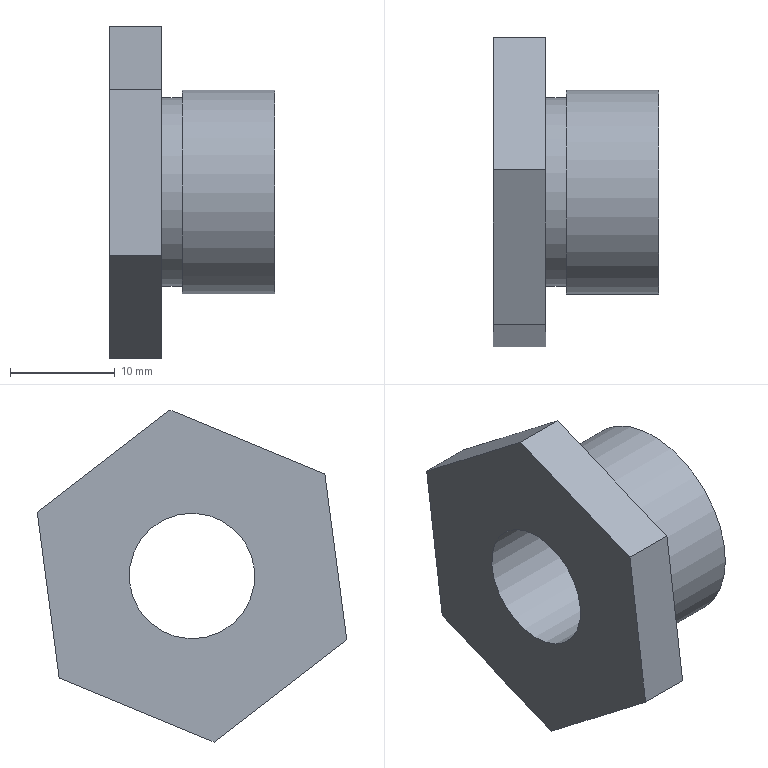Component | NX | LOCK_SLEEVE | 1 solid | 13 faces | box 15.82 x 29.58 x 31.72 mm | volume 4679 mm3 | plane 10 | cylinder 3 | commonest cylinder face diameters 19.5 x1 12 x1 18 x1
STEP:
#1=CARTESIAN_POINT('',(0.,0.,0.));
#2=DIRECTION('',(0.,0.,1.));
#3=DIRECTION('',(1.,0.,0.));
#4=AXIS2_PLACEMENT_3D('',#1,#2,#3);
#5=CARTESIAN_POINT('',(83.182,-9.011,-3.723));
#6=VERTEX_POINT('',#5);
#7=CARTESIAN_POINT('',(83.182,0.,0.));
#8=DIRECTION('',(1.,0.,0.));
#9=DIRECTION('',(0.,-0.9242,-0.3818));
#10=AXIS2_PLACEMENT_3D('',#7,#8,#9);
#11=CIRCLE('',#10,9.75);
#12=CARTESIAN_POINT('',(92.,0.,0.));
#13=DIRECTION('',(-1.,0.,0.));
#14=DIRECTION('',(0.,0.9242,0.3818));
#15=AXIS2_PLACEMENT_3D('',#12,#13,#14);
#16=CYLINDRICAL_SURFACE('',#15,9.75);
#17=CARTESIAN_POINT('',(9.425,8.818));
#18=DIRECTION('',(-1.,0.));
#19=VECTOR('',#18,1.);
#20=LINE('',#17,#19);
#21=(GEOMETRIC_REPRESENTATION_CONTEXT(2)PARAMETRIC_REPRESENTATION_CONTEXT()REPRESENTATION_CONTEXT('',''));
#22=DEFINITIONAL_REPRESENTATION('',(#20),#21);
#23=PCURVE('',#16,#22);
#24=CARTESIAN_POINT('',(83.182,0.,0.));
#25=DIRECTION('',(1.,0.,0.));
#26=DIRECTION('',(0.,-0.9242,-0.3818));
#27=AXIS2_PLACEMENT_3D('',#24,#25,#26);
#28=PLANE('',#27);
#29=CARTESIAN_POINT('',(0.,0.));
#30=DIRECTION('',(1.,0.));
#31=AXIS2_PLACEMENT_2D('',#29,#30);
#32=CIRCLE('',#31,9.75);
#33=(GEOMETRIC_REPRESENTATION_CONTEXT(2)PARAMETRIC_REPRESENTATION_CONTEXT()REPRESENTATION_CONTEXT('',''));
#34=DEFINITIONAL_REPRESENTATION('',(#32),#33);
#35=PCURVE('',#28,#34);
#36=SURFACE_CURVE('',#11,(#23,#35),.PCURVE_S1.);
#37=EDGE_CURVE('',#6,#6,#36,.T.);
#38=ORIENTED_EDGE('',*,*,#37,.T.);
#39=CARTESIAN_POINT('',(92.,-9.011,-3.723));
#40=VERTEX_POINT('',#39);
#41=CARTESIAN_POINT('',(92.,-9.011,-3.723));
#42=CARTESIAN_POINT('',(83.182,-9.011,-3.723));
#43=B_SPLINE_CURVE_WITH_KNOTS('',1,(#41,#42),.UNSPECIFIED.,.F.,.F.,(2,2),(0.,8.818),.PIECEWISE_BEZIER_KNOTS.);
#44=CARTESIAN_POINT('',(3.142,0.));
#45=DIRECTION('',(0.,1.));
#46=VECTOR('',#45,1.);
#47=LINE('',#44,#46);
#48=(GEOMETRIC_REPRESENTATION_CONTEXT(2)PARAMETRIC_REPRESENTATION_CONTEXT()REPRESENTATION_CONTEXT('',''));
#49=DEFINITIONAL_REPRESENTATION('',(#47),#48);
#50=PCURVE('',#16,#49);
#51=CARTESIAN_POINT('',(9.425,0.));
#52=DIRECTION('',(0.,1.));
#53=VECTOR('',#52,1.);
#54=LINE('',#51,#53);
#55=(GEOMETRIC_REPRESENTATION_CONTEXT(2)PARAMETRIC_REPRESENTATION_CONTEXT()REPRESENTATION_CONTEXT('',''));
#56=DEFINITIONAL_REPRESENTATION('',(#54),#55);
#57=PCURVE('',#16,#56);
#58=SEAM_CURVE('',#43,(#50,#57),.PCURVE_S1.);
#59=EDGE_CURVE('',#40,#6,#58,.T.);
#60=ORIENTED_EDGE('',*,*,#59,.F.);
#61=CARTESIAN_POINT('',(92.,0.,0.));
#62=DIRECTION('',(1.,0.,0.));
#63=DIRECTION('',(0.,-0.9242,-0.3818));
#64=AXIS2_PLACEMENT_3D('',#61,#62,#63);
#65=CIRCLE('',#64,9.75);
#66=CARTESIAN_POINT('',(9.425,0.));
#67=DIRECTION('',(-1.,0.));
#68=VECTOR('',#67,1.);
#69=LINE('',#66,#68);
#70=(GEOMETRIC_REPRESENTATION_CONTEXT(2)PARAMETRIC_REPRESENTATION_CONTEXT()REPRESENTATION_CONTEXT('',''));
#71=DEFINITIONAL_REPRESENTATION('',(#69),#70);
#72=PCURVE('',#16,#71);
#73=CARTESIAN_POINT('',(92.,0.,0.));
#74=DIRECTION('',(1.,0.,0.));
#75=DIRECTION('',(0.,-0.9242,-0.3818));
#76=AXIS2_PLACEMENT_3D('',#73,#74,#75);
#77=PLANE('',#76);
#78=CARTESIAN_POINT('',(0.,0.));
#79=DIRECTION('',(1.,0.));
#80=AXIS2_PLACEMENT_2D('',#78,#79);
#81=CIRCLE('',#80,9.75);
#82=(GEOMETRIC_REPRESENTATION_CONTEXT(2)PARAMETRIC_REPRESENTATION_CONTEXT()REPRESENTATION_CONTEXT('',''));
#83=DEFINITIONAL_REPRESENTATION('',(#81),#82);
#84=PCURVE('',#77,#83);
#85=SURFACE_CURVE('',#65,(#72,#84),.PCURVE_S1.);
#86=EDGE_CURVE('',#40,#40,#85,.T.);
#87=ORIENTED_EDGE('',*,*,#86,.F.);
#88=ORIENTED_EDGE('',*,*,#59,.T.);
#89=EDGE_LOOP('',(#38,#60,#87,#88));
#90=FACE_BOUND('',#89,.T.);
#91=ADVANCED_FACE('',(#90),#16,.T.);
#92=CARTESIAN_POINT('',(92.,-5.545,-2.291));
#93=VERTEX_POINT('',#92);
#94=CARTESIAN_POINT('',(92.,0.,0.));
#95=DIRECTION('',(-1.,0.,0.));
#96=DIRECTION('',(0.,-0.9242,-0.3818));
#97=AXIS2_PLACEMENT_3D('',#94,#95,#96);
#98=CIRCLE('',#97,6.);
#99=CARTESIAN_POINT('',(6.,0.));
#100=CARTESIAN_POINT('',(6.,-10.392));
#101=CARTESIAN_POINT('',(-3.,-5.196));
#102=CARTESIAN_POINT('',(-12.,-0.));
#103=CARTESIAN_POINT('',(-3.,5.196));
#104=CARTESIAN_POINT('',(6.,10.392));
#105=CARTESIAN_POINT('',(6.,0.));
#106=(BOUNDED_CURVE()B_SPLINE_CURVE(2,(#99,#100,#101,#102,#103,#104,#105),.UNSPECIFIED.,.T.,.F.)B_SPLINE_CURVE_WITH_KNOTS((1,2,2,2,2,1),(-2.094,0.,2.094,4.189,6.283,8.378),.UNSPECIFIED.)CURVE()GEOMETRIC_REPRESENTATION_ITEM()RATIONAL_B_SPLINE_CURVE((1.,0.5,1.,0.5,1.,0.5,1.))REPRESENTATION_ITEM(''));
#107=(GEOMETRIC_REPRESENTATION_CONTEXT(2)PARAMETRIC_REPRESENTATION_CONTEXT()REPRESENTATION_CONTEXT('',''));
#108=DEFINITIONAL_REPRESENTATION('',(#106),#107);
#109=PCURVE('',#77,#108);
#110=CARTESIAN_POINT('',(102.182,0.,0.));
#111=DIRECTION('',(-1.,0.,0.));
#112=DIRECTION('',(0.,0.9242,0.3818));
#113=AXIS2_PLACEMENT_3D('',#110,#111,#112);
#114=CYLINDRICAL_SURFACE('',#113,6.);
#115=CARTESIAN_POINT('',(3.142,10.182));
#116=DIRECTION('',(1.,0.));
#117=VECTOR('',#116,1.);
#118=LINE('',#115,#117);
#119=(GEOMETRIC_REPRESENTATION_CONTEXT(2)PARAMETRIC_REPRESENTATION_CONTEXT()REPRESENTATION_CONTEXT('',''));
#120=DEFINITIONAL_REPRESENTATION('',(#118),#119);
#121=PCURVE('',#114,#120);
#122=SURFACE_CURVE('',#98,(#109,#121),.PCURVE_S1.);
#123=EDGE_CURVE('',#93,#93,#122,.T.);
#124=ORIENTED_EDGE('',*,*,#123,.T.);
#125=EDGE_LOOP('',(#124));
#126=FACE_BOUND('',#125,.T.);
#127=ORIENTED_EDGE('',*,*,#86,.T.);
#128=EDGE_LOOP('',(#127));
#129=FACE_BOUND('',#128,.T.);
#130=ADVANCED_FACE('',(#126,#129),#77,.T.);
#131=CARTESIAN_POINT('',(81.182,14.788,6.11));
#132=VERTEX_POINT('',#131);
#133=CARTESIAN_POINT('',(81.182,2.103,15.861));
#134=VERTEX_POINT('',#133);
#135=CARTESIAN_POINT('',(81.182,14.788,6.11));
#136=DIRECTION('',(0.,-0.7928,0.6095));
#137=VECTOR('',#136,1.);
#138=LINE('',#135,#137);
#139=CARTESIAN_POINT('',(76.182,14.788,6.11));
#140=DIRECTION('',(0.,0.6095,0.7928));
#141=DIRECTION('',(0.,-0.7928,0.6095));
#142=AXIS2_PLACEMENT_3D('',#139,#140,#141);
#143=PLANE('',#142);
#144=CARTESIAN_POINT('',(0.,5.));
#145=DIRECTION('',(1.,0.));
#146=VECTOR('',#145,1.);
#147=LINE('',#144,#146);
#148=(GEOMETRIC_REPRESENTATION_CONTEXT(2)PARAMETRIC_REPRESENTATION_CONTEXT()REPRESENTATION_CONTEXT('',''));
#149=DEFINITIONAL_REPRESENTATION('',(#147),#148);
#150=PCURVE('',#143,#149);
#151=CARTESIAN_POINT('',(81.182,0.,0.));
#152=DIRECTION('',(1.,0.,0.));
#153=DIRECTION('',(0.,-0.9242,-0.3818));
#154=AXIS2_PLACEMENT_3D('',#151,#152,#153);
#155=PLANE('',#154);
#156=CARTESIAN_POINT('',(-16.,0.));
#157=DIRECTION('',(0.5,-0.866));
#158=VECTOR('',#157,1.);
#159=LINE('',#156,#158);
#160=(GEOMETRIC_REPRESENTATION_CONTEXT(2)PARAMETRIC_REPRESENTATION_CONTEXT()REPRESENTATION_CONTEXT('',''));
#161=DEFINITIONAL_REPRESENTATION('',(#159),#160);
#162=PCURVE('',#155,#161);
#163=SURFACE_CURVE('',#138,(#150,#162),.PCURVE_S1.);
#164=EDGE_CURVE('',#132,#134,#163,.T.);
#165=ORIENTED_EDGE('',*,*,#164,.F.);
#166=CARTESIAN_POINT('',(76.182,14.788,6.11));
#167=VERTEX_POINT('',#166);
#168=CARTESIAN_POINT('',(76.182,14.788,6.11));
#169=DIRECTION('',(1.,0.,0.));
#170=VECTOR('',#169,1.);
#171=LINE('',#168,#170);
#172=CARTESIAN_POINT('',(0.,0.));
#173=DIRECTION('',(0.,1.));
#174=VECTOR('',#173,1.);
#175=LINE('',#172,#174);
#176=(GEOMETRIC_REPRESENTATION_CONTEXT(2)PARAMETRIC_REPRESENTATION_CONTEXT()REPRESENTATION_CONTEXT('',''));
#177=DEFINITIONAL_REPRESENTATION('',(#175),#176);
#178=PCURVE('',#143,#177);
#179=CARTESIAN_POINT('',(76.182,12.685,-9.752));
#180=DIRECTION('',(0.,0.9913,-0.1314));
#181=DIRECTION('',(0.,0.1314,0.9913));
#182=AXIS2_PLACEMENT_3D('',#179,#180,#181);
#183=PLANE('',#182);
#184=CARTESIAN_POINT('',(16.,0.));
#185=DIRECTION('',(0.,1.));
#186=VECTOR('',#185,1.);
#187=LINE('',#184,#186);
#188=(GEOMETRIC_REPRESENTATION_CONTEXT(2)PARAMETRIC_REPRESENTATION_CONTEXT()REPRESENTATION_CONTEXT('',''));
#189=DEFINITIONAL_REPRESENTATION('',(#187),#188);
#190=PCURVE('',#183,#189);
#191=SURFACE_CURVE('',#171,(#178,#190),.PCURVE_S1.);
#192=EDGE_CURVE('',#167,#132,#191,.T.);
#193=ORIENTED_EDGE('',*,*,#192,.F.);
#194=CARTESIAN_POINT('',(76.182,2.103,15.861));
#195=VERTEX_POINT('',#194);
#196=CARTESIAN_POINT('',(76.182,14.788,6.11));
#197=DIRECTION('',(0.,-0.7928,0.6095));
#198=VECTOR('',#197,1.);
#199=LINE('',#196,#198);
#200=CARTESIAN_POINT('',(0.,0.));
#201=DIRECTION('',(1.,0.));
#202=VECTOR('',#201,1.);
#203=LINE('',#200,#202);
#204=(GEOMETRIC_REPRESENTATION_CONTEXT(2)PARAMETRIC_REPRESENTATION_CONTEXT()REPRESENTATION_CONTEXT('',''));
#205=DEFINITIONAL_REPRESENTATION('',(#203),#204);
#206=PCURVE('',#143,#205);
#207=CARTESIAN_POINT('',(76.182,0.,0.));
#208=DIRECTION('',(1.,0.,0.));
#209=DIRECTION('',(0.,-0.9242,-0.3818));
#210=AXIS2_PLACEMENT_3D('',#207,#208,#209);
#211=PLANE('',#210);
#212=CARTESIAN_POINT('',(-16.,0.));
#213=DIRECTION('',(0.5,-0.866));
#214=VECTOR('',#213,1.);
#215=LINE('',#212,#214);
#216=(GEOMETRIC_REPRESENTATION_CONTEXT(2)PARAMETRIC_REPRESENTATION_CONTEXT()REPRESENTATION_CONTEXT('',''));
#217=DEFINITIONAL_REPRESENTATION('',(#215),#216);
#218=PCURVE('',#211,#217);
#219=SURFACE_CURVE('',#199,(#206,#218),.PCURVE_S1.);
#220=EDGE_CURVE('',#167,#195,#219,.T.);
#221=ORIENTED_EDGE('',*,*,#220,.T.);
#222=CARTESIAN_POINT('',(76.182,2.103,15.861));
#223=DIRECTION('',(1.,0.,0.));
#224=VECTOR('',#223,1.);
#225=LINE('',#222,#224);
#226=CARTESIAN_POINT('',(16.,0.));
#227=DIRECTION('',(0.,1.));
#228=VECTOR('',#227,1.);
#229=LINE('',#226,#228);
#230=(GEOMETRIC_REPRESENTATION_CONTEXT(2)PARAMETRIC_REPRESENTATION_CONTEXT()REPRESENTATION_CONTEXT('',''));
#231=DEFINITIONAL_REPRESENTATION('',(#229),#230);
#232=PCURVE('',#143,#231);
#233=CARTESIAN_POINT('',(76.182,2.103,15.861));
#234=DIRECTION('',(0.,-0.3818,0.9242));
#235=DIRECTION('',(0.,-0.9242,-0.3818));
#236=AXIS2_PLACEMENT_3D('',#233,#234,#235);
#237=PLANE('',#236);
#238=CARTESIAN_POINT('',(0.,0.));
#239=DIRECTION('',(0.,1.));
#240=VECTOR('',#239,1.);
#241=LINE('',#238,#240);
#242=(GEOMETRIC_REPRESENTATION_CONTEXT(2)PARAMETRIC_REPRESENTATION_CONTEXT()REPRESENTATION_CONTEXT('',''));
#243=DEFINITIONAL_REPRESENTATION('',(#241),#242);
#244=PCURVE('',#237,#243);
#245=SURFACE_CURVE('',#225,(#232,#244),.PCURVE_S1.);
#246=EDGE_CURVE('',#195,#134,#245,.T.);
#247=ORIENTED_EDGE('',*,*,#246,.T.);
#248=EDGE_LOOP('',(#165,#193,#221,#247));
#249=FACE_BOUND('',#248,.T.);
#250=ADVANCED_FACE('',(#249),#143,.T.);
#251=CARTESIAN_POINT('',(81.182,-12.685,9.752));
#252=VERTEX_POINT('',#251);
#253=CARTESIAN_POINT('',(81.182,2.103,15.861));
#254=DIRECTION('',(0.,-0.9242,-0.3818));
#255=VECTOR('',#254,1.);
#256=LINE('',#253,#255);
#257=CARTESIAN_POINT('',(0.,5.));
#258=DIRECTION('',(1.,0.));
#259=VECTOR('',#258,1.);
#260=LINE('',#257,#259);
#261=(GEOMETRIC_REPRESENTATION_CONTEXT(2)PARAMETRIC_REPRESENTATION_CONTEXT()REPRESENTATION_CONTEXT('',''));
#262=DEFINITIONAL_REPRESENTATION('',(#260),#261);
#263=PCURVE('',#237,#262);
#264=CARTESIAN_POINT('',(-8.,-13.856));
#265=DIRECTION('',(1.,-0.));
#266=VECTOR('',#265,1.);
#267=LINE('',#264,#266);
#268=(GEOMETRIC_REPRESENTATION_CONTEXT(2)PARAMETRIC_REPRESENTATION_CONTEXT()REPRESENTATION_CONTEXT('',''));
#269=DEFINITIONAL_REPRESENTATION('',(#267),#268);
#270=PCURVE('',#155,#269);
#271=SURFACE_CURVE('',#256,(#263,#270),.PCURVE_S1.);
#272=EDGE_CURVE('',#134,#252,#271,.T.);
#273=ORIENTED_EDGE('',*,*,#272,.F.);
#274=ORIENTED_EDGE('',*,*,#246,.F.);
#275=CARTESIAN_POINT('',(76.182,-12.685,9.752));
#276=VERTEX_POINT('',#275);
#277=CARTESIAN_POINT('',(76.182,2.103,15.861));
#278=DIRECTION('',(0.,-0.9242,-0.3818));
#279=VECTOR('',#278,1.);
#280=LINE('',#277,#279);
#281=CARTESIAN_POINT('',(0.,0.));
#282=DIRECTION('',(1.,0.));
#283=VECTOR('',#282,1.);
#284=LINE('',#281,#283);
#285=(GEOMETRIC_REPRESENTATION_CONTEXT(2)PARAMETRIC_REPRESENTATION_CONTEXT()REPRESENTATION_CONTEXT('',''));
#286=DEFINITIONAL_REPRESENTATION('',(#284),#285);
#287=PCURVE('',#237,#286);
#288=CARTESIAN_POINT('',(-8.,-13.856));
#289=DIRECTION('',(1.,-0.));
#290=VECTOR('',#289,1.);
#291=LINE('',#288,#290);
#292=(GEOMETRIC_REPRESENTATION_CONTEXT(2)PARAMETRIC_REPRESENTATION_CONTEXT()REPRESENTATION_CONTEXT('',''));
#293=DEFINITIONAL_REPRESENTATION('',(#291),#292);
#294=PCURVE('',#211,#293);
#295=SURFACE_CURVE('',#280,(#287,#294),.PCURVE_S1.);
#296=EDGE_CURVE('',#195,#276,#295,.T.);
#297=ORIENTED_EDGE('',*,*,#296,.T.);
#298=CARTESIAN_POINT('',(76.182,-12.685,9.752));
#299=DIRECTION('',(1.,0.,0.));
#300=VECTOR('',#299,1.);
#301=LINE('',#298,#300);
#302=CARTESIAN_POINT('',(16.,0.));
#303=DIRECTION('',(0.,1.));
#304=VECTOR('',#303,1.);
#305=LINE('',#302,#304);
#306=(GEOMETRIC_REPRESENTATION_CONTEXT(2)PARAMETRIC_REPRESENTATION_CONTEXT()REPRESENTATION_CONTEXT('',''));
#307=DEFINITIONAL_REPRESENTATION('',(#305),#306);
#308=PCURVE('',#237,#307);
#309=CARTESIAN_POINT('',(76.182,-12.685,9.752));
#310=DIRECTION('',(0.,-0.9913,0.1314));
#311=DIRECTION('',(0.,-0.1314,-0.9913));
#312=AXIS2_PLACEMENT_3D('',#309,#310,#311);
#313=PLANE('',#312);
#314=CARTESIAN_POINT('',(0.,0.));
#315=DIRECTION('',(0.,1.));
#316=VECTOR('',#315,1.);
#317=LINE('',#314,#316);
#318=(GEOMETRIC_REPRESENTATION_CONTEXT(2)PARAMETRIC_REPRESENTATION_CONTEXT()REPRESENTATION_CONTEXT('',''));
#319=DEFINITIONAL_REPRESENTATION('',(#317),#318);
#320=PCURVE('',#313,#319);
#321=SURFACE_CURVE('',#301,(#308,#320),.PCURVE_S1.);
#322=EDGE_CURVE('',#276,#252,#321,.T.);
#323=ORIENTED_EDGE('',*,*,#322,.T.);
#324=EDGE_LOOP('',(#273,#274,#297,#323));
#325=FACE_BOUND('',#324,.T.);
#326=ADVANCED_FACE('',(#325),#237,.T.);
#327=CARTESIAN_POINT('',(81.182,-14.788,-6.11));
#328=VERTEX_POINT('',#327);
#329=CARTESIAN_POINT('',(81.182,-12.685,9.752));
#330=DIRECTION('',(0.,-0.1314,-0.9913));
#331=VECTOR('',#330,1.);
#332=LINE('',#329,#331);
#333=CARTESIAN_POINT('',(0.,5.));
#334=DIRECTION('',(1.,0.));
#335=VECTOR('',#334,1.);
#336=LINE('',#333,#335);
#337=(GEOMETRIC_REPRESENTATION_CONTEXT(2)PARAMETRIC_REPRESENTATION_CONTEXT()REPRESENTATION_CONTEXT('',''));
#338=DEFINITIONAL_REPRESENTATION('',(#336),#337);
#339=PCURVE('',#313,#338);
#340=CARTESIAN_POINT('',(8.,-13.856));
#341=DIRECTION('',(0.5,0.866));
#342=VECTOR('',#341,1.);
#343=LINE('',#340,#342);
#344=(GEOMETRIC_REPRESENTATION_CONTEXT(2)PARAMETRIC_REPRESENTATION_CONTEXT()REPRESENTATION_CONTEXT('',''));
#345=DEFINITIONAL_REPRESENTATION('',(#343),#344);
#346=PCURVE('',#155,#345);
#347=SURFACE_CURVE('',#332,(#339,#346),.PCURVE_S1.);
#348=EDGE_CURVE('',#252,#328,#347,.T.);
#349=ORIENTED_EDGE('',*,*,#348,.F.);
#350=ORIENTED_EDGE('',*,*,#322,.F.);
#351=CARTESIAN_POINT('',(76.182,-14.788,-6.11));
#352=VERTEX_POINT('',#351);
#353=CARTESIAN_POINT('',(76.182,-12.685,9.752));
#354=DIRECTION('',(0.,-0.1314,-0.9913));
#355=VECTOR('',#354,1.);
#356=LINE('',#353,#355);
#357=CARTESIAN_POINT('',(0.,0.));
#358=DIRECTION('',(1.,0.));
#359=VECTOR('',#358,1.);
#360=LINE('',#357,#359);
#361=(GEOMETRIC_REPRESENTATION_CONTEXT(2)PARAMETRIC_REPRESENTATION_CONTEXT()REPRESENTATION_CONTEXT('',''));
#362=DEFINITIONAL_REPRESENTATION('',(#360),#361);
#363=PCURVE('',#313,#362);
#364=CARTESIAN_POINT('',(8.,-13.856));
#365=DIRECTION('',(0.5,0.866));
#366=VECTOR('',#365,1.);
#367=LINE('',#364,#366);
#368=(GEOMETRIC_REPRESENTATION_CONTEXT(2)PARAMETRIC_REPRESENTATION_CONTEXT()REPRESENTATION_CONTEXT('',''));
#369=DEFINITIONAL_REPRESENTATION('',(#367),#368);
#370=PCURVE('',#211,#369);
#371=SURFACE_CURVE('',#356,(#363,#370),.PCURVE_S1.);
#372=EDGE_CURVE('',#276,#352,#371,.T.);
#373=ORIENTED_EDGE('',*,*,#372,.T.);
#374=CARTESIAN_POINT('',(76.182,-14.788,-6.11));
#375=DIRECTION('',(1.,0.,0.));
#376=VECTOR('',#375,1.);
#377=LINE('',#374,#376);
#378=CARTESIAN_POINT('',(16.,0.));
#379=DIRECTION('',(0.,1.));
#380=VECTOR('',#379,1.);
#381=LINE('',#378,#380);
#382=(GEOMETRIC_REPRESENTATION_CONTEXT(2)PARAMETRIC_REPRESENTATION_CONTEXT()REPRESENTATION_CONTEXT('',''));
#383=DEFINITIONAL_REPRESENTATION('',(#381),#382);
#384=PCURVE('',#313,#383);
#385=CARTESIAN_POINT('',(76.182,-14.788,-6.11));
#386=DIRECTION('',(0.,-0.6095,-0.7928));
#387=DIRECTION('',(0.,0.7928,-0.6095));
#388=AXIS2_PLACEMENT_3D('',#385,#386,#387);
#389=PLANE('',#388);
#390=CARTESIAN_POINT('',(-0.,0.));
#391=DIRECTION('',(0.,1.));
#392=VECTOR('',#391,1.);
#393=LINE('',#390,#392);
#394=(GEOMETRIC_REPRESENTATION_CONTEXT(2)PARAMETRIC_REPRESENTATION_CONTEXT()REPRESENTATION_CONTEXT('',''));
#395=DEFINITIONAL_REPRESENTATION('',(#393),#394);
#396=PCURVE('',#389,#395);
#397=SURFACE_CURVE('',#377,(#384,#396),.PCURVE_S1.);
#398=EDGE_CURVE('',#352,#328,#397,.T.);
#399=ORIENTED_EDGE('',*,*,#398,.T.);
#400=EDGE_LOOP('',(#349,#350,#373,#399));
#401=FACE_BOUND('',#400,.T.);
#402=ADVANCED_FACE('',(#401),#313,.T.);
#403=CARTESIAN_POINT('',(81.182,-2.103,-15.861));
#404=VERTEX_POINT('',#403);
#405=CARTESIAN_POINT('',(81.182,-14.788,-6.11));
#406=DIRECTION('',(0.,0.7928,-0.6095));
#407=VECTOR('',#406,1.);
#408=LINE('',#405,#407);
#409=CARTESIAN_POINT('',(0.,5.));
#410=DIRECTION('',(1.,0.));
#411=VECTOR('',#410,1.);
#412=LINE('',#409,#411);
#413=(GEOMETRIC_REPRESENTATION_CONTEXT(2)PARAMETRIC_REPRESENTATION_CONTEXT()REPRESENTATION_CONTEXT('',''));
#414=DEFINITIONAL_REPRESENTATION('',(#412),#413);
#415=PCURVE('',#389,#414);
#416=CARTESIAN_POINT('',(16.,-0.));
#417=DIRECTION('',(-0.5,0.866));
#418=VECTOR('',#417,1.);
#419=LINE('',#416,#418);
#420=(GEOMETRIC_REPRESENTATION_CONTEXT(2)PARAMETRIC_REPRESENTATION_CONTEXT()REPRESENTATION_CONTEXT('',''));
#421=DEFINITIONAL_REPRESENTATION('',(#419),#420);
#422=PCURVE('',#155,#421);
#423=SURFACE_CURVE('',#408,(#415,#422),.PCURVE_S1.);
#424=EDGE_CURVE('',#328,#404,#423,.T.);
#425=ORIENTED_EDGE('',*,*,#424,.F.);
#426=ORIENTED_EDGE('',*,*,#398,.F.);
#427=CARTESIAN_POINT('',(76.182,-2.103,-15.861));
#428=VERTEX_POINT('',#427);
#429=CARTESIAN_POINT('',(76.182,-14.788,-6.11));
#430=DIRECTION('',(0.,0.7928,-0.6095));
#431=VECTOR('',#430,1.);
#432=LINE('',#429,#431);
#433=CARTESIAN_POINT('',(0.,0.));
#434=DIRECTION('',(1.,0.));
#435=VECTOR('',#434,1.);
#436=LINE('',#433,#435);
#437=(GEOMETRIC_REPRESENTATION_CONTEXT(2)PARAMETRIC_REPRESENTATION_CONTEXT()REPRESENTATION_CONTEXT('',''));
#438=DEFINITIONAL_REPRESENTATION('',(#436),#437);
#439=PCURVE('',#389,#438);
#440=CARTESIAN_POINT('',(16.,-0.));
#441=DIRECTION('',(-0.5,0.866));
#442=VECTOR('',#441,1.);
#443=LINE('',#440,#442);
#444=(GEOMETRIC_REPRESENTATION_CONTEXT(2)PARAMETRIC_REPRESENTATION_CONTEXT()REPRESENTATION_CONTEXT('',''));
#445=DEFINITIONAL_REPRESENTATION('',(#443),#444);
#446=PCURVE('',#211,#445);
#447=SURFACE_CURVE('',#432,(#439,#446),.PCURVE_S1.);
#448=EDGE_CURVE('',#352,#428,#447,.T.);
#449=ORIENTED_EDGE('',*,*,#448,.T.);
#450=CARTESIAN_POINT('',(76.182,-2.103,-15.861));
#451=DIRECTION('',(1.,0.,0.));
#452=VECTOR('',#451,1.);
#453=LINE('',#450,#452);
#454=CARTESIAN_POINT('',(16.,0.));
#455=DIRECTION('',(0.,1.));
#456=VECTOR('',#455,1.);
#457=LINE('',#454,#456);
#458=(GEOMETRIC_REPRESENTATION_CONTEXT(2)PARAMETRIC_REPRESENTATION_CONTEXT()REPRESENTATION_CONTEXT('',''));
#459=DEFINITIONAL_REPRESENTATION('',(#457),#458);
#460=PCURVE('',#389,#459);
#461=CARTESIAN_POINT('',(76.182,-2.103,-15.861));
#462=DIRECTION('',(0.,0.3818,-0.9242));
#463=DIRECTION('',(0.,0.9242,0.3818));
#464=AXIS2_PLACEMENT_3D('',#461,#462,#463);
#465=PLANE('',#464);
#466=CARTESIAN_POINT('',(0.,0.));
#467=DIRECTION('',(0.,1.));
#468=VECTOR('',#467,1.);
#469=LINE('',#466,#468);
#470=(GEOMETRIC_REPRESENTATION_CONTEXT(2)PARAMETRIC_REPRESENTATION_CONTEXT()REPRESENTATION_CONTEXT('',''));
#471=DEFINITIONAL_REPRESENTATION('',(#469),#470);
#472=PCURVE('',#465,#471);
#473=SURFACE_CURVE('',#453,(#460,#472),.PCURVE_S1.);
#474=EDGE_CURVE('',#428,#404,#473,.T.);
#475=ORIENTED_EDGE('',*,*,#474,.T.);
#476=EDGE_LOOP('',(#425,#426,#449,#475));
#477=FACE_BOUND('',#476,.T.);
#478=ADVANCED_FACE('',(#477),#389,.T.);
#479=CARTESIAN_POINT('',(81.182,12.685,-9.752));
#480=VERTEX_POINT('',#479);
#481=CARTESIAN_POINT('',(81.182,-2.103,-15.861));
#482=DIRECTION('',(0.,0.9242,0.3818));
#483=VECTOR('',#482,1.);
#484=LINE('',#481,#483);
#485=CARTESIAN_POINT('',(0.,5.));
#486=DIRECTION('',(1.,0.));
#487=VECTOR('',#486,1.);
#488=LINE('',#485,#487);
#489=(GEOMETRIC_REPRESENTATION_CONTEXT(2)PARAMETRIC_REPRESENTATION_CONTEXT()REPRESENTATION_CONTEXT('',''));
#490=DEFINITIONAL_REPRESENTATION('',(#488),#489);
#491=PCURVE('',#465,#490);
#492=CARTESIAN_POINT('',(8.,13.856));
#493=DIRECTION('',(-1.,0.));
#494=VECTOR('',#493,1.);
#495=LINE('',#492,#494);
#496=(GEOMETRIC_REPRESENTATION_CONTEXT(2)PARAMETRIC_REPRESENTATION_CONTEXT()REPRESENTATION_CONTEXT('',''));
#497=DEFINITIONAL_REPRESENTATION('',(#495),#496);
#498=PCURVE('',#155,#497);
#499=SURFACE_CURVE('',#484,(#491,#498),.PCURVE_S1.);
#500=EDGE_CURVE('',#404,#480,#499,.T.);
#501=ORIENTED_EDGE('',*,*,#500,.F.);
#502=ORIENTED_EDGE('',*,*,#474,.F.);
#503=CARTESIAN_POINT('',(76.182,12.685,-9.752));
#504=VERTEX_POINT('',#503);
#505=CARTESIAN_POINT('',(76.182,-2.103,-15.861));
#506=DIRECTION('',(0.,0.9242,0.3818));
#507=VECTOR('',#506,1.);
#508=LINE('',#505,#507);
#509=CARTESIAN_POINT('',(0.,0.));
#510=DIRECTION('',(1.,0.));
#511=VECTOR('',#510,1.);
#512=LINE('',#509,#511);
#513=(GEOMETRIC_REPRESENTATION_CONTEXT(2)PARAMETRIC_REPRESENTATION_CONTEXT()REPRESENTATION_CONTEXT('',''));
#514=DEFINITIONAL_REPRESENTATION('',(#512),#513);
#515=PCURVE('',#465,#514);
#516=CARTESIAN_POINT('',(8.,13.856));
#517=DIRECTION('',(-1.,0.));
#518=VECTOR('',#517,1.);
#519=LINE('',#516,#518);
#520=(GEOMETRIC_REPRESENTATION_CONTEXT(2)PARAMETRIC_REPRESENTATION_CONTEXT()REPRESENTATION_CONTEXT('',''));
#521=DEFINITIONAL_REPRESENTATION('',(#519),#520);
#522=PCURVE('',#211,#521);
#523=SURFACE_CURVE('',#508,(#515,#522),.PCURVE_S1.);
#524=EDGE_CURVE('',#428,#504,#523,.T.);
#525=ORIENTED_EDGE('',*,*,#524,.T.);
#526=CARTESIAN_POINT('',(76.182,12.685,-9.752));
#527=DIRECTION('',(1.,0.,0.));
#528=VECTOR('',#527,1.);
#529=LINE('',#526,#528);
#530=CARTESIAN_POINT('',(16.,0.));
#531=DIRECTION('',(0.,1.));
#532=VECTOR('',#531,1.);
#533=LINE('',#530,#532);
#534=(GEOMETRIC_REPRESENTATION_CONTEXT(2)PARAMETRIC_REPRESENTATION_CONTEXT()REPRESENTATION_CONTEXT('',''));
#535=DEFINITIONAL_REPRESENTATION('',(#533),#534);
#536=PCURVE('',#465,#535);
#537=CARTESIAN_POINT('',(0.,0.));
#538=DIRECTION('',(0.,1.));
#539=VECTOR('',#538,1.);
#540=LINE('',#537,#539);
#541=(GEOMETRIC_REPRESENTATION_CONTEXT(2)PARAMETRIC_REPRESENTATION_CONTEXT()REPRESENTATION_CONTEXT('',''));
#542=DEFINITIONAL_REPRESENTATION('',(#540),#541);
#543=PCURVE('',#183,#542);
#544=SURFACE_CURVE('',#529,(#536,#543),.PCURVE_S1.);
#545=EDGE_CURVE('',#504,#480,#544,.T.);
#546=ORIENTED_EDGE('',*,*,#545,.T.);
#547=EDGE_LOOP('',(#501,#502,#525,#546));
#548=FACE_BOUND('',#547,.T.);
#549=ADVANCED_FACE('',(#548),#465,.T.);
#550=CARTESIAN_POINT('',(81.182,12.685,-9.752));
#551=DIRECTION('',(0.,0.1314,0.9913));
#552=VECTOR('',#551,1.);
#553=LINE('',#550,#552);
#554=CARTESIAN_POINT('',(0.,5.));
#555=DIRECTION('',(1.,0.));
#556=VECTOR('',#555,1.);
#557=LINE('',#554,#556);
#558=(GEOMETRIC_REPRESENTATION_CONTEXT(2)PARAMETRIC_REPRESENTATION_CONTEXT()REPRESENTATION_CONTEXT('',''));
#559=DEFINITIONAL_REPRESENTATION('',(#557),#558);
#560=PCURVE('',#183,#559);
#561=CARTESIAN_POINT('',(-8.,13.856));
#562=DIRECTION('',(-0.5,-0.866));
#563=VECTOR('',#562,1.);
#564=LINE('',#561,#563);
#565=(GEOMETRIC_REPRESENTATION_CONTEXT(2)PARAMETRIC_REPRESENTATION_CONTEXT()REPRESENTATION_CONTEXT('',''));
#566=DEFINITIONAL_REPRESENTATION('',(#564),#565);
#567=PCURVE('',#155,#566);
#568=SURFACE_CURVE('',#553,(#560,#567),.PCURVE_S1.);
#569=EDGE_CURVE('',#480,#132,#568,.T.);
#570=ORIENTED_EDGE('',*,*,#569,.F.);
#571=ORIENTED_EDGE('',*,*,#545,.F.);
#572=CARTESIAN_POINT('',(76.182,12.685,-9.752));
#573=DIRECTION('',(0.,0.1314,0.9913));
#574=VECTOR('',#573,1.);
#575=LINE('',#572,#574);
#576=CARTESIAN_POINT('',(0.,0.));
#577=DIRECTION('',(1.,0.));
#578=VECTOR('',#577,1.);
#579=LINE('',#576,#578);
#580=(GEOMETRIC_REPRESENTATION_CONTEXT(2)PARAMETRIC_REPRESENTATION_CONTEXT()REPRESENTATION_CONTEXT('',''));
#581=DEFINITIONAL_REPRESENTATION('',(#579),#580);
#582=PCURVE('',#183,#581);
#583=CARTESIAN_POINT('',(-8.,13.856));
#584=DIRECTION('',(-0.5,-0.866));
#585=VECTOR('',#584,1.);
#586=LINE('',#583,#585);
#587=(GEOMETRIC_REPRESENTATION_CONTEXT(2)PARAMETRIC_REPRESENTATION_CONTEXT()REPRESENTATION_CONTEXT('',''));
#588=DEFINITIONAL_REPRESENTATION('',(#586),#587);
#589=PCURVE('',#211,#588);
#590=SURFACE_CURVE('',#575,(#582,#589),.PCURVE_S1.);
#591=EDGE_CURVE('',#504,#167,#590,.T.);
#592=ORIENTED_EDGE('',*,*,#591,.T.);
#593=ORIENTED_EDGE('',*,*,#192,.T.);
#594=EDGE_LOOP('',(#570,#571,#592,#593));
#595=FACE_BOUND('',#594,.T.);
#596=ADVANCED_FACE('',(#595),#183,.T.);
#597=CARTESIAN_POINT('',(76.182,-5.545,-2.291));
#598=VERTEX_POINT('',#597);
#599=CARTESIAN_POINT('',(76.182,0.,0.));
#600=DIRECTION('',(-1.,0.,0.));
#601=DIRECTION('',(0.,-0.9242,-0.3818));
#602=AXIS2_PLACEMENT_3D('',#599,#600,#601);
#603=CIRCLE('',#602,6.);
#604=CARTESIAN_POINT('',(6.,0.));
#605=CARTESIAN_POINT('',(6.,-10.392));
#606=CARTESIAN_POINT('',(-3.,-5.196));
#607=CARTESIAN_POINT('',(-12.,-0.));
#608=CARTESIAN_POINT('',(-3.,5.196));
#609=CARTESIAN_POINT('',(6.,10.392));
#610=CARTESIAN_POINT('',(6.,0.));
#611=(BOUNDED_CURVE()B_SPLINE_CURVE(2,(#604,#605,#606,#607,#608,#609,#610),.UNSPECIFIED.,.T.,.F.)B_SPLINE_CURVE_WITH_KNOTS((1,2,2,2,2,1),(-2.094,0.,2.094,4.189,6.283,8.378),.UNSPECIFIED.)CURVE()GEOMETRIC_REPRESENTATION_ITEM()RATIONAL_B_SPLINE_CURVE((1.,0.5,1.,0.5,1.,0.5,1.))REPRESENTATION_ITEM(''));
#612=(GEOMETRIC_REPRESENTATION_CONTEXT(2)PARAMETRIC_REPRESENTATION_CONTEXT()REPRESENTATION_CONTEXT('',''));
#613=DEFINITIONAL_REPRESENTATION('',(#611),#612);
#614=PCURVE('',#211,#613);
#615=CARTESIAN_POINT('',(3.142,26.));
#616=DIRECTION('',(1.,0.));
#617=VECTOR('',#616,1.);
#618=LINE('',#615,#617);
#619=(GEOMETRIC_REPRESENTATION_CONTEXT(2)PARAMETRIC_REPRESENTATION_CONTEXT()REPRESENTATION_CONTEXT('',''));
#620=DEFINITIONAL_REPRESENTATION('',(#618),#619);
#621=PCURVE('',#114,#620);
#622=SURFACE_CURVE('',#603,(#614,#621),.PCURVE_S1.);
#623=EDGE_CURVE('',#598,#598,#622,.T.);
#624=ORIENTED_EDGE('',*,*,#623,.F.);
#625=EDGE_LOOP('',(#624));
#626=FACE_BOUND('',#625,.T.);
#627=ORIENTED_EDGE('',*,*,#220,.F.);
#628=ORIENTED_EDGE('',*,*,#591,.F.);
#629=ORIENTED_EDGE('',*,*,#524,.F.);
#630=ORIENTED_EDGE('',*,*,#448,.F.);
#631=ORIENTED_EDGE('',*,*,#372,.F.);
#632=ORIENTED_EDGE('',*,*,#296,.F.);
#633=EDGE_LOOP('',(#627,#628,#629,#630,#631,#632));
#634=FACE_BOUND('',#633,.T.);
#635=ADVANCED_FACE('',(#626,#634),#211,.F.);
#636=ORIENTED_EDGE('',*,*,#164,.T.);
#637=ORIENTED_EDGE('',*,*,#272,.T.);
#638=ORIENTED_EDGE('',*,*,#348,.T.);
#639=ORIENTED_EDGE('',*,*,#424,.T.);
#640=ORIENTED_EDGE('',*,*,#500,.T.);
#641=ORIENTED_EDGE('',*,*,#569,.T.);
#642=EDGE_LOOP('',(#636,#637,#638,#639,#640,#641));
#643=FACE_BOUND('',#642,.T.);
#644=CARTESIAN_POINT('',(81.182,-8.318,-3.437));
#645=VERTEX_POINT('',#644);
#646=CARTESIAN_POINT('',(81.182,0.,0.));
#647=DIRECTION('',(1.,0.,0.));
#648=DIRECTION('',(0.,-0.9242,-0.3818));
#649=AXIS2_PLACEMENT_3D('',#646,#647,#648);
#650=CIRCLE('',#649,9.);
#651=CARTESIAN_POINT('',(0.,0.));
#652=DIRECTION('',(1.,0.));
#653=AXIS2_PLACEMENT_2D('',#651,#652);
#654=CIRCLE('',#653,9.);
#655=(GEOMETRIC_REPRESENTATION_CONTEXT(2)PARAMETRIC_REPRESENTATION_CONTEXT()REPRESENTATION_CONTEXT('',''));
#656=DEFINITIONAL_REPRESENTATION('',(#654),#655);
#657=PCURVE('',#155,#656);
#658=CARTESIAN_POINT('',(83.182,0.,0.));
#659=DIRECTION('',(-1.,0.,0.));
#660=DIRECTION('',(0.,0.9242,0.3818));
#661=AXIS2_PLACEMENT_3D('',#658,#659,#660);
#662=CYLINDRICAL_SURFACE('',#661,9.);
#663=CARTESIAN_POINT('',(9.425,2.));
#664=DIRECTION('',(-1.,0.));
#665=VECTOR('',#664,1.);
#666=LINE('',#663,#665);
#667=(GEOMETRIC_REPRESENTATION_CONTEXT(2)PARAMETRIC_REPRESENTATION_CONTEXT()REPRESENTATION_CONTEXT('',''));
#668=DEFINITIONAL_REPRESENTATION('',(#666),#667);
#669=PCURVE('',#662,#668);
#670=SURFACE_CURVE('',#650,(#657,#669),.PCURVE_S1.);
#671=EDGE_CURVE('',#645,#645,#670,.T.);
#672=ORIENTED_EDGE('',*,*,#671,.F.);
#673=EDGE_LOOP('',(#672));
#674=FACE_BOUND('',#673,.T.);
#675=ADVANCED_FACE('',(#643,#674),#155,.T.);
#676=ORIENTED_EDGE('',*,*,#123,.T.);
#677=CARTESIAN_POINT('',(92.,-5.545,-2.291));
#678=CARTESIAN_POINT('',(76.182,-5.545,-2.291));
#679=B_SPLINE_CURVE_WITH_KNOTS('',1,(#677,#678),.UNSPECIFIED.,.F.,.F.,(2,2),(10.182,26.),.PIECEWISE_BEZIER_KNOTS.);
#680=CARTESIAN_POINT('',(9.425,0.));
#681=DIRECTION('',(0.,1.));
#682=VECTOR('',#681,1.);
#683=LINE('',#680,#682);
#684=(GEOMETRIC_REPRESENTATION_CONTEXT(2)PARAMETRIC_REPRESENTATION_CONTEXT()REPRESENTATION_CONTEXT('',''));
#685=DEFINITIONAL_REPRESENTATION('',(#683),#684);
#686=PCURVE('',#114,#685);
#687=CARTESIAN_POINT('',(3.142,0.));
#688=DIRECTION('',(0.,1.));
#689=VECTOR('',#688,1.);
#690=LINE('',#687,#689);
#691=(GEOMETRIC_REPRESENTATION_CONTEXT(2)PARAMETRIC_REPRESENTATION_CONTEXT()REPRESENTATION_CONTEXT('',''));
#692=DEFINITIONAL_REPRESENTATION('',(#690),#691);
#693=PCURVE('',#114,#692);
#694=SEAM_CURVE('',#679,(#686,#693),.PCURVE_S1.);
#695=EDGE_CURVE('',#93,#598,#694,.T.);
#696=ORIENTED_EDGE('',*,*,#695,.T.);
#697=ORIENTED_EDGE('',*,*,#623,.F.);
#698=ORIENTED_EDGE('',*,*,#695,.F.);
#699=EDGE_LOOP('',(#676,#696,#697,#698));
#700=FACE_BOUND('',#699,.F.);
#701=ADVANCED_FACE('',(#700),#114,.F.);
#702=CARTESIAN_POINT('',(83.182,-8.318,-3.437));
#703=VERTEX_POINT('',#702);
#704=CARTESIAN_POINT('',(83.182,0.,0.));
#705=DIRECTION('',(-1.,0.,0.));
#706=DIRECTION('',(0.,-0.9242,-0.3818));
#707=AXIS2_PLACEMENT_3D('',#704,#705,#706);
#708=CIRCLE('',#707,9.);
#709=CARTESIAN_POINT('',(9.,0.));
#710=CARTESIAN_POINT('',(9.,-15.588));
#711=CARTESIAN_POINT('',(-4.5,-7.794));
#712=CARTESIAN_POINT('',(-18.,-0.));
#713=CARTESIAN_POINT('',(-4.5,7.794));
#714=CARTESIAN_POINT('',(9.,15.588));
#715=CARTESIAN_POINT('',(9.,0.));
#716=(BOUNDED_CURVE()B_SPLINE_CURVE(2,(#709,#710,#711,#712,#713,#714,#715),.UNSPECIFIED.,.T.,.F.)B_SPLINE_CURVE_WITH_KNOTS((1,2,2,2,2,1),(-2.094,0.,2.094,4.189,6.283,8.378),.UNSPECIFIED.)CURVE()GEOMETRIC_REPRESENTATION_ITEM()RATIONAL_B_SPLINE_CURVE((1.,0.5,1.,0.5,1.,0.5,1.))REPRESENTATION_ITEM(''));
#717=(GEOMETRIC_REPRESENTATION_CONTEXT(2)PARAMETRIC_REPRESENTATION_CONTEXT()REPRESENTATION_CONTEXT('',''));
#718=DEFINITIONAL_REPRESENTATION('',(#716),#717);
#719=PCURVE('',#28,#718);
#720=CARTESIAN_POINT('',(3.142,0.));
#721=DIRECTION('',(1.,0.));
#722=VECTOR('',#721,1.);
#723=LINE('',#720,#722);
#724=(GEOMETRIC_REPRESENTATION_CONTEXT(2)PARAMETRIC_REPRESENTATION_CONTEXT()REPRESENTATION_CONTEXT('',''));
#725=DEFINITIONAL_REPRESENTATION('',(#723),#724);
#726=PCURVE('',#662,#725);
#727=SURFACE_CURVE('',#708,(#719,#726),.PCURVE_S1.);
#728=EDGE_CURVE('',#703,#703,#727,.T.);
#729=ORIENTED_EDGE('',*,*,#728,.F.);
#730=EDGE_LOOP('',(#729));
#731=FACE_BOUND('',#730,.T.);
#732=ORIENTED_EDGE('',*,*,#37,.F.);
#733=EDGE_LOOP('',(#732));
#734=FACE_BOUND('',#733,.T.);
#735=ADVANCED_FACE('',(#731,#734),#28,.F.);
#736=ORIENTED_EDGE('',*,*,#728,.T.);
#737=CARTESIAN_POINT('',(83.182,-8.318,-3.437));
#738=CARTESIAN_POINT('',(81.182,-8.318,-3.437));
#739=B_SPLINE_CURVE_WITH_KNOTS('',1,(#737,#738),.UNSPECIFIED.,.F.,.F.,(2,2),(0.,2.),.PIECEWISE_BEZIER_KNOTS.);
#740=CARTESIAN_POINT('',(9.425,0.));
#741=DIRECTION('',(0.,1.));
#742=VECTOR('',#741,1.);
#743=LINE('',#740,#742);
#744=(GEOMETRIC_REPRESENTATION_CONTEXT(2)PARAMETRIC_REPRESENTATION_CONTEXT()REPRESENTATION_CONTEXT('',''));
#745=DEFINITIONAL_REPRESENTATION('',(#743),#744);
#746=PCURVE('',#662,#745);
#747=CARTESIAN_POINT('',(3.142,0.));
#748=DIRECTION('',(0.,1.));
#749=VECTOR('',#748,1.);
#750=LINE('',#747,#749);
#751=(GEOMETRIC_REPRESENTATION_CONTEXT(2)PARAMETRIC_REPRESENTATION_CONTEXT()REPRESENTATION_CONTEXT('',''));
#752=DEFINITIONAL_REPRESENTATION('',(#750),#751);
#753=PCURVE('',#662,#752);
#754=SEAM_CURVE('',#739,(#746,#753),.PCURVE_S1.);
#755=EDGE_CURVE('',#703,#645,#754,.T.);
#756=ORIENTED_EDGE('',*,*,#755,.T.);
#757=ORIENTED_EDGE('',*,*,#671,.T.);
#758=ORIENTED_EDGE('',*,*,#755,.F.);
#759=EDGE_LOOP('',(#736,#756,#757,#758));
#760=FACE_BOUND('',#759,.T.);
#761=ADVANCED_FACE('',(#760),#662,.T.);
#762=CLOSED_SHELL('',(#91,#130,#250,#326,#402,#478,#549,#596,#635,#675,#701,#735,#761));
#763=MANIFOLD_SOLID_BREP('',#762);
#764=(LENGTH_UNIT()NAMED_UNIT(*)SI_UNIT(.MILLI.,.METRE.));
#765=UNCERTAINTY_MEASURE_WITH_UNIT(LENGTH_MEASURE(0.000002),#764,'','');
#766=(NAMED_UNIT(*)PLANE_ANGLE_UNIT()SI_UNIT($,.RADIAN.));
#767=(NAMED_UNIT(*)SI_UNIT($,.STERADIAN.)SOLID_ANGLE_UNIT());
#768=(GEOMETRIC_REPRESENTATION_CONTEXT(3)GLOBAL_UNCERTAINTY_ASSIGNED_CONTEXT((#765))GLOBAL_UNIT_ASSIGNED_CONTEXT((#764,#766,#767))REPRESENTATION_CONTEXT('',''));
#769=ADVANCED_BREP_SHAPE_REPRESENTATION('',(#4,#763),#768);